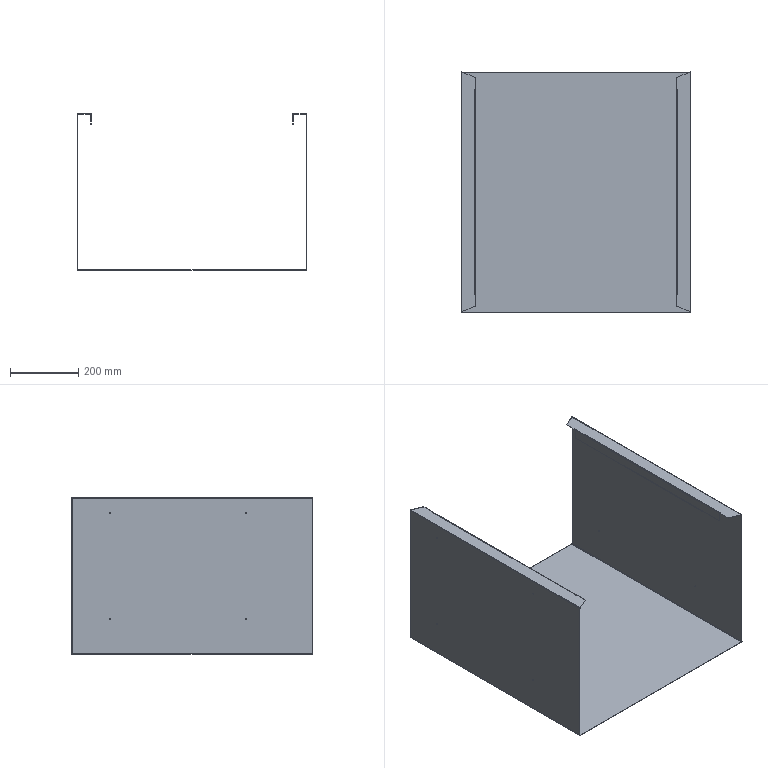Component | SolidWorks | PC-CAJ-P08-1_PM-CAJ-P34-1 | 1 solid | 99 faces | volume 1204734 mm3 | plane 71 | cylinder 28 | commonest cylinder face diameters 3 x22 1 x6 | material Plain Carbon Steel